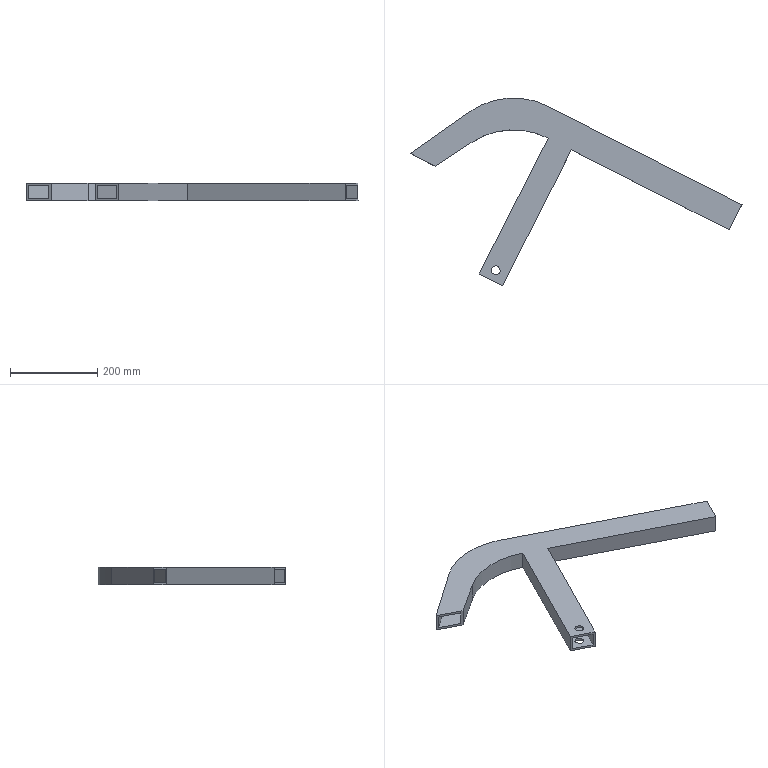Component | SolidWorks | FrameAssemblyDrawing11111-1_PartFrameCorner-1 | 1 solid | 30 faces | box 762.68 x 431.5 x 40 mm | volume 1076455 mm3 | plane 22 | cylinder 8 | commonest cylinder face diameters 20 x4 350 x2 360 x1 340 x1
STEP:
#1=COLOUR_RGB('',0.7922,0.8196,0.9333);
#2=FILL_AREA_STYLE_COLOUR('',#1);
#3=FILL_AREA_STYLE('',(#2));
#4=SURFACE_STYLE_FILL_AREA(#3);
#5=SURFACE_SIDE_STYLE('',(#4));
#6=SURFACE_STYLE_USAGE(.BOTH.,#5);
#7=PRESENTATION_STYLE_ASSIGNMENT((#6));
#8=CARTESIAN_POINT('',(-46.867,-24.103,40.983));
#9=VERTEX_POINT('',#8);
#10=CARTESIAN_POINT('',(-46.165,-24.459,40.983));
#11=VERTEX_POINT('',#10);
#12=CARTESIAN_POINT('',(-46.516,-24.281,40.983));
#13=DIRECTION('',(-0.,-0.,1.));
#14=DIRECTION('',(0.892,-0.4521,-0.));
#15=AXIS2_PLACEMENT_3D('',#12,#13,#14);
#16=CIRCLE('',#15,0.3937);
#17=EDGE_CURVE('',#9,#11,#16,.T.);
#18=ORIENTED_EDGE('',*,*,#17,.F.);
#19=CARTESIAN_POINT('',(-46.867,-24.103,41.18));
#20=VERTEX_POINT('',#19);
#21=CARTESIAN_POINT('',(-46.867,-24.103,40.983));
#22=DIRECTION('',(-0.,-0.,1.));
#23=VECTOR('',#22,39.37);
#24=LINE('',#21,#23);
#25=EDGE_CURVE('',#9,#20,#24,.T.);
#26=ORIENTED_EDGE('',*,*,#25,.T.);
#27=CARTESIAN_POINT('',(-46.165,-24.459,41.18));
#28=VERTEX_POINT('',#27);
#29=CARTESIAN_POINT('',(-46.516,-24.281,41.18));
#30=DIRECTION('',(-0.,-0.,1.));
#31=DIRECTION('',(0.892,-0.4521,-0.));
#32=AXIS2_PLACEMENT_3D('',#29,#30,#31);
#33=CIRCLE('',#32,0.3937);
#34=EDGE_CURVE('',#20,#28,#33,.T.);
#35=ORIENTED_EDGE('',*,*,#34,.T.);
#36=CARTESIAN_POINT('',(-46.165,-24.459,40.983));
#37=DIRECTION('',(-0.,-0.,1.));
#38=VECTOR('',#37,39.37);
#39=LINE('',#36,#38);
#40=EDGE_CURVE('',#11,#28,#39,.T.);
#41=ORIENTED_EDGE('',*,*,#40,.F.);
#42=EDGE_LOOP('',(#18,#26,#35,#41));
#43=FACE_OUTER_BOUND('',#42,.T.);
#44=CARTESIAN_POINT('',(-46.516,-24.281,40.983));
#45=DIRECTION('',(-0.,-0.,1.));
#46=DIRECTION('',(0.892,-0.4521,-0.));
#47=AXIS2_PLACEMENT_3D('',#44,#45,#46);
#48=CYLINDRICAL_SURFACE('',#47,0.3937);
#49=ADVANCED_FACE('',(#43),#48,.F.);
#50=CARTESIAN_POINT('',(-46.165,-24.459,42.361));
#51=VERTEX_POINT('',#50);
#52=CARTESIAN_POINT('',(-46.867,-24.103,42.361));
#53=VERTEX_POINT('',#52);
#54=CARTESIAN_POINT('',(-46.516,-24.281,42.361));
#55=DIRECTION('',(0.,0.,-1.));
#56=DIRECTION('',(-0.892,0.4521,0.));
#57=AXIS2_PLACEMENT_3D('',#54,#55,#56);
#58=CIRCLE('',#57,0.3937);
#59=EDGE_CURVE('',#51,#53,#58,.T.);
#60=ORIENTED_EDGE('',*,*,#59,.T.);
#61=CARTESIAN_POINT('',(-46.867,-24.103,42.558));
#62=VERTEX_POINT('',#61);
#63=CARTESIAN_POINT('',(-46.867,-24.103,40.983));
#64=DIRECTION('',(-0.,-0.,1.));
#65=VECTOR('',#64,39.37);
#66=LINE('',#63,#65);
#67=EDGE_CURVE('',#53,#62,#66,.T.);
#68=ORIENTED_EDGE('',*,*,#67,.T.);
#69=CARTESIAN_POINT('',(-46.165,-24.459,42.558));
#70=VERTEX_POINT('',#69);
#71=CARTESIAN_POINT('',(-46.516,-24.281,42.558));
#72=DIRECTION('',(-0.,-0.,1.));
#73=DIRECTION('',(0.892,-0.4521,-0.));
#74=AXIS2_PLACEMENT_3D('',#71,#72,#73);
#75=CIRCLE('',#74,0.3937);
#76=EDGE_CURVE('',#62,#70,#75,.T.);
#77=ORIENTED_EDGE('',*,*,#76,.T.);
#78=CARTESIAN_POINT('',(-46.165,-24.459,40.983));
#79=DIRECTION('',(-0.,-0.,1.));
#80=VECTOR('',#79,39.37);
#81=LINE('',#78,#80);
#82=EDGE_CURVE('',#51,#70,#81,.T.);
#83=ORIENTED_EDGE('',*,*,#82,.F.);
#84=EDGE_LOOP('',(#60,#68,#77,#83));
#85=FACE_OUTER_BOUND('',#84,.T.);
#86=CARTESIAN_POINT('',(-46.516,-24.281,40.983));
#87=DIRECTION('',(-0.,-0.,1.));
#88=DIRECTION('',(0.892,-0.4521,-0.));
#89=AXIS2_PLACEMENT_3D('',#86,#87,#88);
#90=CYLINDRICAL_SURFACE('',#89,0.3937);
#91=ADVANCED_FACE('',(#85),#90,.F.);
#92=CARTESIAN_POINT('',(-39.678,-13.402,40.983));
#93=VERTEX_POINT('',#92);
#94=CARTESIAN_POINT('',(-39.678,-13.402,42.558));
#95=VERTEX_POINT('',#94);
#96=CARTESIAN_POINT('',(-39.678,-13.402,40.983));
#97=DIRECTION('',(-0.,-0.,1.));
#98=VECTOR('',#97,39.37);
#99=LINE('',#96,#98);
#100=EDGE_CURVE('',#93,#95,#99,.T.);
#101=ORIENTED_EDGE('',*,*,#100,.F.);
#102=CARTESIAN_POINT('',(-25.406,-20.636,40.983));
#103=VERTEX_POINT('',#102);
#104=CARTESIAN_POINT('',(-41.785,-12.334,40.983));
#105=DIRECTION('',(0.892,-0.4521,-0.));
#106=VECTOR('',#105,39.37);
#107=LINE('',#104,#106);
#108=EDGE_CURVE('',#93,#103,#107,.T.);
#109=ORIENTED_EDGE('',*,*,#108,.T.);
#110=CARTESIAN_POINT('',(-25.406,-20.636,42.558));
#111=VERTEX_POINT('',#110);
#112=CARTESIAN_POINT('',(-25.406,-20.636,42.558));
#113=DIRECTION('',(0.,0.,-1.));
#114=VECTOR('',#113,39.37);
#115=LINE('',#112,#114);
#116=EDGE_CURVE('',#111,#103,#115,.T.);
#117=ORIENTED_EDGE('',*,*,#116,.F.);
#118=CARTESIAN_POINT('',(-41.785,-12.334,42.558));
#119=DIRECTION('',(0.892,-0.4521,-0.));
#120=VECTOR('',#119,39.37);
#121=LINE('',#118,#120);
#122=EDGE_CURVE('',#95,#111,#121,.T.);
#123=ORIENTED_EDGE('',*,*,#122,.F.);
#124=EDGE_LOOP('',(#101,#109,#117,#123));
#125=FACE_OUTER_BOUND('',#124,.T.);
#126=CARTESIAN_POINT('',(-41.785,-12.334,42.558));
#127=DIRECTION('',(0.4521,0.892,0.));
#128=DIRECTION('',(-0.892,0.4521,0.));
#129=AXIS2_PLACEMENT_3D('',#126,#127,#128);
#130=PLANE('',#129);
#131=ADVANCED_FACE('',(#125),#130,.F.);
#132=CARTESIAN_POINT('',(-54.273,-13.723,40.983));
#133=VERTEX_POINT('',#132);
#134=CARTESIAN_POINT('',(-51.991,-14.88,40.983));
#135=VERTEX_POINT('',#134);
#136=CARTESIAN_POINT('',(-54.273,-13.723,40.983));
#137=DIRECTION('',(0.892,-0.4521,-0.));
#138=VECTOR('',#137,39.37);
#139=LINE('',#136,#138);
#140=EDGE_CURVE('',#133,#135,#139,.T.);
#141=ORIENTED_EDGE('',*,*,#140,.T.);
#142=CARTESIAN_POINT('',(-51.991,-14.88,42.558));
#143=VERTEX_POINT('',#142);
#144=CARTESIAN_POINT('',(-51.991,-14.88,42.558));
#145=DIRECTION('',(0.,0.,-1.));
#146=VECTOR('',#145,39.37);
#147=LINE('',#144,#146);
#148=EDGE_CURVE('',#143,#135,#147,.T.);
#149=ORIENTED_EDGE('',*,*,#148,.F.);
#150=CARTESIAN_POINT('',(-54.273,-13.723,42.558));
#151=VERTEX_POINT('',#150);
#152=CARTESIAN_POINT('',(-54.273,-13.723,42.558));
#153=DIRECTION('',(0.892,-0.4521,-0.));
#154=VECTOR('',#153,39.37);
#155=LINE('',#152,#154);
#156=EDGE_CURVE('',#151,#143,#155,.T.);
#157=ORIENTED_EDGE('',*,*,#156,.F.);
#158=CARTESIAN_POINT('',(-54.273,-13.723,42.558));
#159=DIRECTION('',(0.,0.,-1.));
#160=VECTOR('',#159,39.37);
#161=LINE('',#158,#160);
#162=EDGE_CURVE('',#151,#133,#161,.T.);
#163=ORIENTED_EDGE('',*,*,#162,.T.);
#164=EDGE_LOOP('',(#141,#149,#157,#163));
#165=FACE_OUTER_BOUND('',#164,.T.);
#166=CARTESIAN_POINT('',(-54.074,-13.824,41.18));
#167=VERTEX_POINT('',#166);
#168=CARTESIAN_POINT('',(-52.194,-14.777,41.18));
#169=VERTEX_POINT('',#168);
#170=CARTESIAN_POINT('',(-46.077,-17.877,41.18));
#171=DIRECTION('',(0.892,-0.4521,-0.));
#172=VECTOR('',#171,39.37);
#173=LINE('',#170,#172);
#174=EDGE_CURVE('',#167,#169,#173,.T.);
#175=ORIENTED_EDGE('',*,*,#174,.F.);
#176=CARTESIAN_POINT('',(-54.074,-13.824,42.361));
#177=VERTEX_POINT('',#176);
#178=CARTESIAN_POINT('',(-54.074,-13.824,42.558));
#179=DIRECTION('',(0.,0.,-1.));
#180=VECTOR('',#179,39.37);
#181=LINE('',#178,#180);
#182=EDGE_CURVE('',#177,#167,#181,.T.);
#183=ORIENTED_EDGE('',*,*,#182,.F.);
#184=CARTESIAN_POINT('',(-52.194,-14.777,42.361));
#185=VERTEX_POINT('',#184);
#186=CARTESIAN_POINT('',(-46.077,-17.877,42.361));
#187=DIRECTION('',(0.892,-0.4521,-0.));
#188=VECTOR('',#187,39.37);
#189=LINE('',#186,#188);
#190=EDGE_CURVE('',#177,#185,#189,.T.);
#191=ORIENTED_EDGE('',*,*,#190,.T.);
#192=CARTESIAN_POINT('',(-52.194,-14.777,42.558));
#193=DIRECTION('',(0.,0.,-1.));
#194=VECTOR('',#193,39.37);
#195=LINE('',#192,#194);
#196=EDGE_CURVE('',#185,#169,#195,.T.);
#197=ORIENTED_EDGE('',*,*,#196,.T.);
#198=EDGE_LOOP('',(#175,#183,#191,#197));
#199=FACE_BOUND('',#198,.T.);
#200=CARTESIAN_POINT('',(-54.273,-13.723,42.558));
#201=DIRECTION('',(0.4521,0.892,0.));
#202=DIRECTION('',(-0.,-0.,1.));
#203=AXIS2_PLACEMENT_3D('',#200,#201,#202);
#204=PLANE('',#203);
#205=ADVANCED_FACE('',(#165,#199),#204,.F.);
#206=CARTESIAN_POINT('',(-24.247,-18.349,40.983));
#207=VERTEX_POINT('',#206);
#208=CARTESIAN_POINT('',(-24.247,-18.349,40.983));
#209=DIRECTION('',(0.4521,0.892,0.));
#210=VECTOR('',#209,39.37);
#211=LINE('',#208,#210);
#212=EDGE_CURVE('',#103,#207,#211,.T.);
#213=ORIENTED_EDGE('',*,*,#212,.T.);
#214=CARTESIAN_POINT('',(-24.247,-18.349,42.558));
#215=VERTEX_POINT('',#214);
#216=CARTESIAN_POINT('',(-24.247,-18.349,42.558));
#217=DIRECTION('',(0.,0.,-1.));
#218=VECTOR('',#217,39.37);
#219=LINE('',#216,#218);
#220=EDGE_CURVE('',#215,#207,#219,.T.);
#221=ORIENTED_EDGE('',*,*,#220,.F.);
#222=CARTESIAN_POINT('',(-24.247,-18.349,42.558));
#223=DIRECTION('',(0.4521,0.892,0.));
#224=VECTOR('',#223,39.37);
#225=LINE('',#222,#224);
#226=EDGE_CURVE('',#111,#215,#225,.T.);
#227=ORIENTED_EDGE('',*,*,#226,.F.);
#228=ORIENTED_EDGE('',*,*,#116,.T.);
#229=EDGE_LOOP('',(#213,#221,#227,#228));
#230=FACE_OUTER_BOUND('',#229,.T.);
#231=CARTESIAN_POINT('',(-25.317,-20.461,41.18));
#232=VERTEX_POINT('',#231);
#233=CARTESIAN_POINT('',(-24.336,-18.524,41.18));
#234=VERTEX_POINT('',#233);
#235=CARTESIAN_POINT('',(-27.361,-24.494,41.18));
#236=DIRECTION('',(0.4521,0.892,0.));
#237=VECTOR('',#236,39.37);
#238=LINE('',#235,#237);
#239=EDGE_CURVE('',#232,#234,#238,.T.);
#240=ORIENTED_EDGE('',*,*,#239,.F.);
#241=CARTESIAN_POINT('',(-25.317,-20.461,42.361));
#242=VERTEX_POINT('',#241);
#243=CARTESIAN_POINT('',(-25.317,-20.461,42.558));
#244=DIRECTION('',(0.,0.,-1.));
#245=VECTOR('',#244,39.37);
#246=LINE('',#243,#245);
#247=EDGE_CURVE('',#242,#232,#246,.T.);
#248=ORIENTED_EDGE('',*,*,#247,.F.);
#249=CARTESIAN_POINT('',(-24.336,-18.524,42.361));
#250=VERTEX_POINT('',#249);
#251=CARTESIAN_POINT('',(-27.361,-24.494,42.361));
#252=DIRECTION('',(0.4521,0.892,0.));
#253=VECTOR('',#252,39.37);
#254=LINE('',#251,#253);
#255=EDGE_CURVE('',#242,#250,#254,.T.);
#256=ORIENTED_EDGE('',*,*,#255,.T.);
#257=CARTESIAN_POINT('',(-24.336,-18.524,42.558));
#258=DIRECTION('',(0.,0.,-1.));
#259=VECTOR('',#258,39.37);
#260=LINE('',#257,#259);
#261=EDGE_CURVE('',#250,#234,#260,.T.);
#262=ORIENTED_EDGE('',*,*,#261,.T.);
#263=EDGE_LOOP('',(#240,#248,#256,#262));
#264=FACE_BOUND('',#263,.T.);
#265=CARTESIAN_POINT('',(-24.247,-18.349,42.558));
#266=DIRECTION('',(-0.892,0.4521,0.));
#267=DIRECTION('',(-0.,-0.,1.));
#268=AXIS2_PLACEMENT_3D('',#265,#266,#267);
#269=PLANE('',#268);
#270=ADVANCED_FACE('',(#230,#264),#269,.F.);
#271=CARTESIAN_POINT('',(-48.864,-9.946,40.983));
#272=VERTEX_POINT('',#271);
#273=CARTESIAN_POINT('',(-54.273,-13.723,40.983));
#274=DIRECTION('',(-0.8199,-0.5725,-0.));
#275=VECTOR('',#274,39.37);
#276=LINE('',#273,#275);
#277=EDGE_CURVE('',#272,#133,#276,.T.);
#278=ORIENTED_EDGE('',*,*,#277,.T.);
#279=ORIENTED_EDGE('',*,*,#162,.F.);
#280=CARTESIAN_POINT('',(-48.864,-9.946,42.558));
#281=VERTEX_POINT('',#280);
#282=CARTESIAN_POINT('',(-54.273,-13.723,42.558));
#283=DIRECTION('',(-0.8199,-0.5725,-0.));
#284=VECTOR('',#283,39.37);
#285=LINE('',#282,#284);
#286=EDGE_CURVE('',#281,#151,#285,.T.);
#287=ORIENTED_EDGE('',*,*,#286,.F.);
#288=CARTESIAN_POINT('',(-48.864,-9.946,42.558));
#289=DIRECTION('',(0.,0.,-1.));
#290=VECTOR('',#289,39.37);
#291=LINE('',#288,#290);
#292=EDGE_CURVE('',#281,#272,#291,.T.);
#293=ORIENTED_EDGE('',*,*,#292,.T.);
#294=EDGE_LOOP('',(#278,#279,#287,#293));
#295=FACE_OUTER_BOUND('',#294,.T.);
#296=CARTESIAN_POINT('',(-54.273,-13.723,42.558));
#297=DIRECTION('',(0.5725,-0.8199,-0.));
#298=DIRECTION('',(0.8199,0.5725,0.));
#299=AXIS2_PLACEMENT_3D('',#296,#297,#298);
#300=PLANE('',#299);
#301=ADVANCED_FACE('',(#295),#300,.F.);
#302=CARTESIAN_POINT('',(-48.664,-12.71,40.983));
#303=VERTEX_POINT('',#302);
#304=CARTESIAN_POINT('',(-51.991,-14.88,40.983));
#305=DIRECTION('',(0.8375,0.5464,0.));
#306=VECTOR('',#305,39.37);
#307=LINE('',#304,#306);
#308=EDGE_CURVE('',#135,#303,#307,.T.);
#309=ORIENTED_EDGE('',*,*,#308,.T.);
#310=CARTESIAN_POINT('',(-48.664,-12.71,42.558));
#311=VERTEX_POINT('',#310);
#312=CARTESIAN_POINT('',(-48.664,-12.71,42.558));
#313=DIRECTION('',(0.,0.,-1.));
#314=VECTOR('',#313,39.37);
#315=LINE('',#312,#314);
#316=EDGE_CURVE('',#311,#303,#315,.T.);
#317=ORIENTED_EDGE('',*,*,#316,.F.);
#318=CARTESIAN_POINT('',(-51.991,-14.88,42.558));
#319=DIRECTION('',(0.8375,0.5464,0.));
#320=VECTOR('',#319,39.37);
#321=LINE('',#318,#320);
#322=EDGE_CURVE('',#143,#311,#321,.T.);
#323=ORIENTED_EDGE('',*,*,#322,.F.);
#324=ORIENTED_EDGE('',*,*,#148,.T.);
#325=EDGE_LOOP('',(#309,#317,#323,#324));
#326=FACE_OUTER_BOUND('',#325,.T.);
#327=CARTESIAN_POINT('',(-51.991,-14.88,42.558));
#328=DIRECTION('',(-0.5464,0.8375,0.));
#329=DIRECTION('',(-0.8375,-0.5464,-0.));
#330=AXIS2_PLACEMENT_3D('',#327,#328,#329);
#331=PLANE('',#330);
#332=ADVANCED_FACE('',(#326),#331,.F.);
#333=CARTESIAN_POINT('',(-41.785,-12.334,40.983));
#334=VERTEX_POINT('',#333);
#335=CARTESIAN_POINT('',(-44.9,-18.48,40.983));
#336=DIRECTION('',(0.,0.,-1.));
#337=DIRECTION('',(-0.892,0.4521,0.));
#338=AXIS2_PLACEMENT_3D('',#335,#336,#337);
#339=CIRCLE('',#338,6.89);
#340=EDGE_CURVE('',#303,#334,#339,.T.);
#341=ORIENTED_EDGE('',*,*,#340,.T.);
#342=CARTESIAN_POINT('',(-41.785,-12.334,42.558));
#343=VERTEX_POINT('',#342);
#344=CARTESIAN_POINT('',(-41.785,-12.334,42.558));
#345=DIRECTION('',(0.,0.,-1.));
#346=VECTOR('',#345,39.37);
#347=LINE('',#344,#346);
#348=EDGE_CURVE('',#343,#334,#347,.T.);
#349=ORIENTED_EDGE('',*,*,#348,.F.);
#350=CARTESIAN_POINT('',(-44.9,-18.48,42.558));
#351=DIRECTION('',(0.,0.,-1.));
#352=DIRECTION('',(-0.892,0.4521,0.));
#353=AXIS2_PLACEMENT_3D('',#350,#351,#352);
#354=CIRCLE('',#353,6.89);
#355=EDGE_CURVE('',#311,#343,#354,.T.);
#356=ORIENTED_EDGE('',*,*,#355,.F.);
#357=ORIENTED_EDGE('',*,*,#316,.T.);
#358=EDGE_LOOP('',(#341,#349,#356,#357));
#359=FACE_OUTER_BOUND('',#358,.T.);
#360=CARTESIAN_POINT('',(-44.9,-18.48,42.558));
#361=DIRECTION('',(0.,0.,-1.));
#362=DIRECTION('',(-0.892,0.4521,0.));
#363=AXIS2_PLACEMENT_3D('',#360,#361,#362);
#364=CYLINDRICAL_SURFACE('',#363,6.89);
#365=ADVANCED_FACE('',(#359),#364,.F.);
#366=CARTESIAN_POINT('',(-41.805,-9.449,40.983));
#367=VERTEX_POINT('',#366);
#368=CARTESIAN_POINT('',(-41.805,-9.449,40.983));
#369=DIRECTION('',(-0.892,0.4521,0.));
#370=VECTOR('',#369,39.37);
#371=LINE('',#368,#370);
#372=EDGE_CURVE('',#207,#367,#371,.T.);
#373=ORIENTED_EDGE('',*,*,#372,.T.);
#374=CARTESIAN_POINT('',(-41.805,-9.449,42.558));
#375=VERTEX_POINT('',#374);
#376=CARTESIAN_POINT('',(-41.805,-9.449,42.558));
#377=DIRECTION('',(0.,0.,-1.));
#378=VECTOR('',#377,39.37);
#379=LINE('',#376,#378);
#380=EDGE_CURVE('',#375,#367,#379,.T.);
#381=ORIENTED_EDGE('',*,*,#380,.F.);
#382=CARTESIAN_POINT('',(-41.805,-9.449,42.558));
#383=DIRECTION('',(-0.892,0.4521,0.));
#384=VECTOR('',#383,39.37);
#385=LINE('',#382,#384);
#386=EDGE_CURVE('',#215,#375,#385,.T.);
#387=ORIENTED_EDGE('',*,*,#386,.F.);
#388=ORIENTED_EDGE('',*,*,#220,.T.);
#389=EDGE_LOOP('',(#373,#381,#387,#388));
#390=FACE_OUTER_BOUND('',#389,.T.);
#391=CARTESIAN_POINT('',(-41.805,-9.449,42.558));
#392=DIRECTION('',(-0.4521,-0.892,-0.));
#393=DIRECTION('',(0.,0.,-1.));
#394=AXIS2_PLACEMENT_3D('',#391,#392,#393);
#395=PLANE('',#394);
#396=ADVANCED_FACE('',(#390),#395,.F.);
#397=CARTESIAN_POINT('',(-44.92,-15.595,40.983));
#398=DIRECTION('',(-0.,-0.,1.));
#399=DIRECTION('',(-0.892,0.4521,0.));
#400=AXIS2_PLACEMENT_3D('',#397,#398,#399);
#401=CIRCLE('',#400,6.89);
#402=EDGE_CURVE('',#367,#272,#401,.T.);
#403=ORIENTED_EDGE('',*,*,#402,.T.);
#404=ORIENTED_EDGE('',*,*,#292,.F.);
#405=CARTESIAN_POINT('',(-44.92,-15.595,42.558));
#406=DIRECTION('',(-0.,-0.,1.));
#407=DIRECTION('',(-0.892,0.4521,0.));
#408=AXIS2_PLACEMENT_3D('',#405,#406,#407);
#409=CIRCLE('',#408,6.89);
#410=EDGE_CURVE('',#375,#281,#409,.T.);
#411=ORIENTED_EDGE('',*,*,#410,.F.);
#412=ORIENTED_EDGE('',*,*,#380,.T.);
#413=EDGE_LOOP('',(#403,#404,#411,#412));
#414=FACE_OUTER_BOUND('',#413,.T.);
#415=CARTESIAN_POINT('',(-44.92,-15.595,42.558));
#416=DIRECTION('',(0.,0.,-1.));
#417=DIRECTION('',(-0.892,0.4521,0.));
#418=AXIS2_PLACEMENT_3D('',#415,#416,#417);
#419=CYLINDRICAL_SURFACE('',#418,6.89);
#420=ADVANCED_FACE('',(#414),#419,.T.);
#421=CARTESIAN_POINT('',(-46.516,-24.281,42.558));
#422=DIRECTION('',(-0.,-0.,1.));
#423=DIRECTION('',(0.892,-0.4521,-0.));
#424=AXIS2_PLACEMENT_3D('',#421,#422,#423);
#425=CIRCLE('',#424,0.3937);
#426=EDGE_CURVE('',#70,#62,#425,.T.);
#427=ORIENTED_EDGE('',*,*,#426,.F.);
#428=ORIENTED_EDGE('',*,*,#76,.F.);
#429=EDGE_LOOP('',(#427,#428));
#430=FACE_BOUND('',#429,.T.);
#431=ORIENTED_EDGE('',*,*,#286,.T.);
#432=ORIENTED_EDGE('',*,*,#156,.T.);
#433=ORIENTED_EDGE('',*,*,#322,.T.);
#434=ORIENTED_EDGE('',*,*,#355,.T.);
#435=CARTESIAN_POINT('',(-48.015,-24.625,42.558));
#436=VERTEX_POINT('',#435);
#437=CARTESIAN_POINT('',(-48.015,-24.625,42.558));
#438=DIRECTION('',(0.4521,0.892,0.));
#439=VECTOR('',#438,39.37);
#440=LINE('',#437,#439);
#441=EDGE_CURVE('',#436,#343,#440,.T.);
#442=ORIENTED_EDGE('',*,*,#441,.F.);
#443=CARTESIAN_POINT('',(-45.908,-25.693,42.558));
#444=VERTEX_POINT('',#443);
#445=CARTESIAN_POINT('',(-48.015,-24.625,42.558));
#446=DIRECTION('',(-0.892,0.4521,0.));
#447=VECTOR('',#446,39.37);
#448=LINE('',#445,#447);
#449=EDGE_CURVE('',#444,#436,#448,.T.);
#450=ORIENTED_EDGE('',*,*,#449,.F.);
#451=CARTESIAN_POINT('',(-45.908,-25.693,42.558));
#452=DIRECTION('',(0.4521,0.892,0.));
#453=VECTOR('',#452,39.37);
#454=LINE('',#451,#453);
#455=EDGE_CURVE('',#444,#95,#454,.T.);
#456=ORIENTED_EDGE('',*,*,#455,.T.);
#457=ORIENTED_EDGE('',*,*,#122,.T.);
#458=ORIENTED_EDGE('',*,*,#226,.T.);
#459=ORIENTED_EDGE('',*,*,#386,.T.);
#460=ORIENTED_EDGE('',*,*,#410,.T.);
#461=EDGE_LOOP('',(#431,#432,#433,#434,#442,#450,#456,#457,#458,#459,#460));
#462=FACE_OUTER_BOUND('',#461,.T.);
#463=CARTESIAN_POINT('',(-44.92,-15.595,42.558));
#464=DIRECTION('',(0.,0.,-1.));
#465=DIRECTION('',(-0.892,0.4521,0.));
#466=AXIS2_PLACEMENT_3D('',#463,#464,#465);
#467=PLANE('',#466);
#468=ADVANCED_FACE('',(#430,#462),#467,.F.);
#469=CARTESIAN_POINT('',(-46.516,-24.281,40.983));
#470=DIRECTION('',(-0.,-0.,1.));
#471=DIRECTION('',(0.892,-0.4521,-0.));
#472=AXIS2_PLACEMENT_3D('',#469,#470,#471);
#473=CIRCLE('',#472,0.3937);
#474=EDGE_CURVE('',#11,#9,#473,.T.);
#475=ORIENTED_EDGE('',*,*,#474,.T.);
#476=ORIENTED_EDGE('',*,*,#17,.T.);
#477=EDGE_LOOP('',(#475,#476));
#478=FACE_BOUND('',#477,.T.);
#479=ORIENTED_EDGE('',*,*,#277,.F.);
#480=ORIENTED_EDGE('',*,*,#402,.F.);
#481=ORIENTED_EDGE('',*,*,#372,.F.);
#482=ORIENTED_EDGE('',*,*,#212,.F.);
#483=ORIENTED_EDGE('',*,*,#108,.F.);
#484=CARTESIAN_POINT('',(-45.908,-25.693,40.983));
#485=VERTEX_POINT('',#484);
#486=CARTESIAN_POINT('',(-45.908,-25.693,40.983));
#487=DIRECTION('',(0.4521,0.892,0.));
#488=VECTOR('',#487,39.37);
#489=LINE('',#486,#488);
#490=EDGE_CURVE('',#485,#93,#489,.T.);
#491=ORIENTED_EDGE('',*,*,#490,.F.);
#492=CARTESIAN_POINT('',(-48.015,-24.625,40.983));
#493=VERTEX_POINT('',#492);
#494=CARTESIAN_POINT('',(-48.015,-24.625,40.983));
#495=DIRECTION('',(0.892,-0.4521,-0.));
#496=VECTOR('',#495,39.37);
#497=LINE('',#494,#496);
#498=EDGE_CURVE('',#493,#485,#497,.T.);
#499=ORIENTED_EDGE('',*,*,#498,.F.);
#500=CARTESIAN_POINT('',(-48.015,-24.625,40.983));
#501=DIRECTION('',(0.4521,0.892,0.));
#502=VECTOR('',#501,39.37);
#503=LINE('',#500,#502);
#504=EDGE_CURVE('',#493,#334,#503,.T.);
#505=ORIENTED_EDGE('',*,*,#504,.T.);
#506=ORIENTED_EDGE('',*,*,#340,.F.);
#507=ORIENTED_EDGE('',*,*,#308,.F.);
#508=ORIENTED_EDGE('',*,*,#140,.F.);
#509=EDGE_LOOP('',(#479,#480,#481,#482,#483,#491,#499,#505,#506,#507,#508));
#510=FACE_OUTER_BOUND('',#509,.T.);
#511=CARTESIAN_POINT('',(-44.92,-15.595,40.983));
#512=DIRECTION('',(0.,0.,-1.));
#513=DIRECTION('',(-0.892,0.4521,0.));
#514=AXIS2_PLACEMENT_3D('',#511,#512,#513);
#515=PLANE('',#514);
#516=ADVANCED_FACE('',(#478,#510),#515,.T.);
#517=CARTESIAN_POINT('',(-48.752,-10.107,41.18));
#518=VERTEX_POINT('',#517);
#519=CARTESIAN_POINT('',(-48.752,-10.107,41.18));
#520=DIRECTION('',(-0.8199,-0.5725,-0.));
#521=VECTOR('',#520,39.37);
#522=LINE('',#519,#521);
#523=EDGE_CURVE('',#518,#167,#522,.T.);
#524=ORIENTED_EDGE('',*,*,#523,.F.);
#525=CARTESIAN_POINT('',(-48.752,-10.107,42.361));
#526=VERTEX_POINT('',#525);
#527=CARTESIAN_POINT('',(-48.752,-10.107,42.558));
#528=DIRECTION('',(0.,0.,-1.));
#529=VECTOR('',#528,39.37);
#530=LINE('',#527,#529);
#531=EDGE_CURVE('',#526,#518,#530,.T.);
#532=ORIENTED_EDGE('',*,*,#531,.F.);
#533=CARTESIAN_POINT('',(-48.752,-10.107,42.361));
#534=DIRECTION('',(-0.8199,-0.5725,-0.));
#535=VECTOR('',#534,39.37);
#536=LINE('',#533,#535);
#537=EDGE_CURVE('',#526,#177,#536,.T.);
#538=ORIENTED_EDGE('',*,*,#537,.T.);
#539=ORIENTED_EDGE('',*,*,#182,.T.);
#540=EDGE_LOOP('',(#524,#532,#538,#539));
#541=FACE_OUTER_BOUND('',#540,.T.);
#542=CARTESIAN_POINT('',(-54.161,-13.884,42.558));
#543=DIRECTION('',(0.5725,-0.8199,-0.));
#544=DIRECTION('',(0.8199,0.5725,0.));
#545=AXIS2_PLACEMENT_3D('',#542,#543,#544);
#546=PLANE('',#545);
#547=ADVANCED_FACE('',(#541),#546,.T.);
#548=CARTESIAN_POINT('',(-48.772,-12.545,41.18));
#549=VERTEX_POINT('',#548);
#550=CARTESIAN_POINT('',(-47.466,-11.692,41.18));
#551=DIRECTION('',(0.8375,0.5464,0.));
#552=VECTOR('',#551,39.37);
#553=LINE('',#550,#552);
#554=EDGE_CURVE('',#169,#549,#553,.T.);
#555=ORIENTED_EDGE('',*,*,#554,.F.);
#556=ORIENTED_EDGE('',*,*,#196,.F.);
#557=CARTESIAN_POINT('',(-48.772,-12.545,42.361));
#558=VERTEX_POINT('',#557);
#559=CARTESIAN_POINT('',(-47.466,-11.692,42.361));
#560=DIRECTION('',(0.8375,0.5464,0.));
#561=VECTOR('',#560,39.37);
#562=LINE('',#559,#561);
#563=EDGE_CURVE('',#185,#558,#562,.T.);
#564=ORIENTED_EDGE('',*,*,#563,.T.);
#565=CARTESIAN_POINT('',(-48.772,-12.545,42.558));
#566=DIRECTION('',(0.,0.,-1.));
#567=VECTOR('',#566,39.37);
#568=LINE('',#565,#567);
#569=EDGE_CURVE('',#558,#549,#568,.T.);
#570=ORIENTED_EDGE('',*,*,#569,.T.);
#571=EDGE_LOOP('',(#555,#556,#564,#570));
#572=FACE_OUTER_BOUND('',#571,.T.);
#573=CARTESIAN_POINT('',(-52.098,-14.715,42.558));
#574=DIRECTION('',(-0.5464,0.8375,0.));
#575=DIRECTION('',(-0.8375,-0.5464,-0.));
#576=AXIS2_PLACEMENT_3D('',#573,#574,#575);
#577=PLANE('',#576);
#578=ADVANCED_FACE('',(#572),#577,.T.);
#579=CARTESIAN_POINT('',(-41.696,-12.159,41.18));
#580=VERTEX_POINT('',#579);
#581=CARTESIAN_POINT('',(-44.9,-18.48,41.18));
#582=DIRECTION('',(0.,0.,-1.));
#583=DIRECTION('',(-0.892,0.4521,0.));
#584=AXIS2_PLACEMENT_3D('',#581,#582,#583);
#585=CIRCLE('',#584,7.087);
#586=EDGE_CURVE('',#549,#580,#585,.T.);
#587=ORIENTED_EDGE('',*,*,#586,.F.);
#588=ORIENTED_EDGE('',*,*,#569,.F.);
#589=CARTESIAN_POINT('',(-41.696,-12.159,42.361));
#590=VERTEX_POINT('',#589);
#591=CARTESIAN_POINT('',(-44.9,-18.48,42.361));
#592=DIRECTION('',(0.,0.,-1.));
#593=DIRECTION('',(-0.892,0.4521,0.));
#594=AXIS2_PLACEMENT_3D('',#591,#592,#593);
#595=CIRCLE('',#594,7.087);
#596=EDGE_CURVE('',#558,#590,#595,.T.);
#597=ORIENTED_EDGE('',*,*,#596,.T.);
#598=CARTESIAN_POINT('',(-41.696,-12.159,42.558));
#599=DIRECTION('',(0.,0.,-1.));
#600=VECTOR('',#599,39.37);
#601=LINE('',#598,#600);
#602=EDGE_CURVE('',#590,#580,#601,.T.);
#603=ORIENTED_EDGE('',*,*,#602,.T.);
#604=EDGE_LOOP('',(#587,#588,#597,#603));
#605=FACE_OUTER_BOUND('',#604,.T.);
#606=CARTESIAN_POINT('',(-44.9,-18.48,42.558));
#607=DIRECTION('',(0.,0.,-1.));
#608=DIRECTION('',(-0.892,0.4521,0.));
#609=AXIS2_PLACEMENT_3D('',#606,#607,#608);
#610=CYLINDRICAL_SURFACE('',#609,7.087);
#611=ADVANCED_FACE('',(#605),#610,.T.);
#612=CARTESIAN_POINT('',(-42.875,-11.561,41.18));
#613=DIRECTION('',(0.892,-0.4521,-0.));
#614=VECTOR('',#613,39.37);
#615=LINE('',#612,#614);
#616=EDGE_CURVE('',#580,#232,#615,.T.);
#617=ORIENTED_EDGE('',*,*,#616,.F.);
#618=ORIENTED_EDGE('',*,*,#602,.F.);
#619=CARTESIAN_POINT('',(-42.875,-11.561,42.361));
#620=DIRECTION('',(0.892,-0.4521,-0.));
#621=VECTOR('',#620,39.37);
#622=LINE('',#619,#621);
#623=EDGE_CURVE('',#590,#242,#622,.T.);
#624=ORIENTED_EDGE('',*,*,#623,.T.);
#625=ORIENTED_EDGE('',*,*,#247,.T.);
#626=EDGE_LOOP('',(#617,#618,#624,#625));
#627=FACE_OUTER_BOUND('',#626,.T.);
#628=CARTESIAN_POINT('',(-41.696,-12.159,42.558));
#629=DIRECTION('',(0.4521,0.892,0.));
#630=DIRECTION('',(-0.892,0.4521,0.));
#631=AXIS2_PLACEMENT_3D('',#628,#629,#630);
#632=PLANE('',#631);
#633=ADVANCED_FACE('',(#627),#632,.T.);
#634=CARTESIAN_POINT('',(-41.894,-9.625,41.18));
#635=VERTEX_POINT('',#634);
#636=CARTESIAN_POINT('',(-41.894,-9.625,41.18));
#637=DIRECTION('',(-0.892,0.4521,0.));
#638=VECTOR('',#637,39.37);
#639=LINE('',#636,#638);
#640=EDGE_CURVE('',#234,#635,#639,.T.);
#641=ORIENTED_EDGE('',*,*,#640,.F.);
#642=ORIENTED_EDGE('',*,*,#261,.F.);
#643=CARTESIAN_POINT('',(-41.894,-9.625,42.361));
#644=VERTEX_POINT('',#643);
#645=CARTESIAN_POINT('',(-41.894,-9.625,42.361));
#646=DIRECTION('',(-0.892,0.4521,0.));
#647=VECTOR('',#646,39.37);
#648=LINE('',#645,#647);
#649=EDGE_CURVE('',#250,#644,#648,.T.);
#650=ORIENTED_EDGE('',*,*,#649,.T.);
#651=CARTESIAN_POINT('',(-41.894,-9.625,42.558));
#652=DIRECTION('',(0.,0.,-1.));
#653=VECTOR('',#652,39.37);
#654=LINE('',#651,#653);
#655=EDGE_CURVE('',#644,#635,#654,.T.);
#656=ORIENTED_EDGE('',*,*,#655,.T.);
#657=EDGE_LOOP('',(#641,#642,#650,#656));
#658=FACE_OUTER_BOUND('',#657,.T.);
#659=CARTESIAN_POINT('',(-41.894,-9.625,42.558));
#660=DIRECTION('',(-0.4521,-0.892,-0.));
#661=DIRECTION('',(0.,0.,-1.));
#662=AXIS2_PLACEMENT_3D('',#659,#660,#661);
#663=PLANE('',#662);
#664=ADVANCED_FACE('',(#658),#663,.T.);
#665=CARTESIAN_POINT('',(-44.92,-15.595,41.18));
#666=DIRECTION('',(-0.,-0.,1.));
#667=DIRECTION('',(-0.892,0.4521,0.));
#668=AXIS2_PLACEMENT_3D('',#665,#666,#667);
#669=CIRCLE('',#668,6.693);
#670=EDGE_CURVE('',#635,#518,#669,.T.);
#671=ORIENTED_EDGE('',*,*,#670,.F.);
#672=ORIENTED_EDGE('',*,*,#655,.F.);
#673=CARTESIAN_POINT('',(-44.92,-15.595,42.361));
#674=DIRECTION('',(-0.,-0.,1.));
#675=DIRECTION('',(-0.892,0.4521,0.));
#676=AXIS2_PLACEMENT_3D('',#673,#674,#675);
#677=CIRCLE('',#676,6.693);
#678=EDGE_CURVE('',#644,#526,#677,.T.);
#679=ORIENTED_EDGE('',*,*,#678,.T.);
#680=ORIENTED_EDGE('',*,*,#531,.T.);
#681=EDGE_LOOP('',(#671,#672,#679,#680));
#682=FACE_OUTER_BOUND('',#681,.T.);
#683=CARTESIAN_POINT('',(-44.92,-15.595,42.558));
#684=DIRECTION('',(0.,0.,-1.));
#685=DIRECTION('',(-0.892,0.4521,0.));
#686=AXIS2_PLACEMENT_3D('',#683,#684,#685);
#687=CYLINDRICAL_SURFACE('',#686,6.693);
#688=ADVANCED_FACE('',(#682),#687,.F.);
#689=ORIENTED_EDGE('',*,*,#537,.F.);
#690=ORIENTED_EDGE('',*,*,#678,.F.);
#691=ORIENTED_EDGE('',*,*,#649,.F.);
#692=ORIENTED_EDGE('',*,*,#255,.F.);
#693=ORIENTED_EDGE('',*,*,#623,.F.);
#694=ORIENTED_EDGE('',*,*,#596,.F.);
#695=ORIENTED_EDGE('',*,*,#563,.F.);
#696=ORIENTED_EDGE('',*,*,#190,.F.);
#697=EDGE_LOOP('',(#689,#690,#691,#692,#693,#694,#695,#696));
#698=FACE_OUTER_BOUND('',#697,.T.);
#699=CARTESIAN_POINT('',(-44.92,-15.595,42.361));
#700=DIRECTION('',(0.,0.,-1.));
#701=DIRECTION('',(-0.892,0.4521,0.));
#702=AXIS2_PLACEMENT_3D('',#699,#700,#701);
#703=PLANE('',#702);
#704=ADVANCED_FACE('',(#698),#703,.T.);
#705=ORIENTED_EDGE('',*,*,#523,.T.);
#706=ORIENTED_EDGE('',*,*,#174,.T.);
#707=ORIENTED_EDGE('',*,*,#554,.T.);
#708=ORIENTED_EDGE('',*,*,#586,.T.);
#709=ORIENTED_EDGE('',*,*,#616,.T.);
#710=ORIENTED_EDGE('',*,*,#239,.T.);
#711=ORIENTED_EDGE('',*,*,#640,.T.);
#712=ORIENTED_EDGE('',*,*,#670,.T.);
#713=EDGE_LOOP('',(#705,#706,#707,#708,#709,#710,#711,#712));
#714=FACE_OUTER_BOUND('',#713,.T.);
#715=CARTESIAN_POINT('',(-44.92,-15.595,41.18));
#716=DIRECTION('',(0.,0.,-1.));
#717=DIRECTION('',(-0.892,0.4521,0.));
#718=AXIS2_PLACEMENT_3D('',#715,#716,#717);
#719=PLANE('',#718);
#720=ADVANCED_FACE('',(#714),#719,.F.);
#721=CARTESIAN_POINT('',(-48.015,-24.625,40.983));
#722=DIRECTION('',(0.,0.,-1.));
#723=VECTOR('',#722,39.37);
#724=LINE('',#721,#723);
#725=EDGE_CURVE('',#436,#493,#724,.T.);
#726=ORIENTED_EDGE('',*,*,#725,.T.);
#727=ORIENTED_EDGE('',*,*,#498,.T.);
#728=CARTESIAN_POINT('',(-45.908,-25.693,40.983));
#729=DIRECTION('',(-0.,-0.,1.));
#730=VECTOR('',#729,39.37);
#731=LINE('',#728,#730);
#732=EDGE_CURVE('',#485,#444,#731,.T.);
#733=ORIENTED_EDGE('',*,*,#732,.T.);
#734=ORIENTED_EDGE('',*,*,#449,.T.);
#735=EDGE_LOOP('',(#726,#727,#733,#734));
#736=FACE_OUTER_BOUND('',#735,.T.);
#737=CARTESIAN_POINT('',(-47.839,-24.714,42.361));
#738=VERTEX_POINT('',#737);
#739=CARTESIAN_POINT('',(-47.839,-24.714,41.18));
#740=VERTEX_POINT('',#739);
#741=CARTESIAN_POINT('',(-47.839,-24.714,41.18));
#742=DIRECTION('',(0.,0.,-1.));
#743=VECTOR('',#742,39.37);
#744=LINE('',#741,#743);
#745=EDGE_CURVE('',#738,#740,#744,.T.);
#746=ORIENTED_EDGE('',*,*,#745,.F.);
#747=CARTESIAN_POINT('',(-46.083,-25.604,42.361));
#748=VERTEX_POINT('',#747);
#749=CARTESIAN_POINT('',(-47.839,-24.714,42.361));
#750=DIRECTION('',(-0.892,0.4521,0.));
#751=VECTOR('',#750,39.37);
#752=LINE('',#749,#751);
#753=EDGE_CURVE('',#748,#738,#752,.T.);
#754=ORIENTED_EDGE('',*,*,#753,.F.);
#755=CARTESIAN_POINT('',(-46.083,-25.604,41.18));
#756=VERTEX_POINT('',#755);
#757=CARTESIAN_POINT('',(-46.083,-25.604,41.18));
#758=DIRECTION('',(-0.,-0.,1.));
#759=VECTOR('',#758,39.37);
#760=LINE('',#757,#759);
#761=EDGE_CURVE('',#756,#748,#760,.T.);
#762=ORIENTED_EDGE('',*,*,#761,.F.);
#763=CARTESIAN_POINT('',(-47.839,-24.714,41.18));
#764=DIRECTION('',(0.892,-0.4521,-0.));
#765=VECTOR('',#764,39.37);
#766=LINE('',#763,#765);
#767=EDGE_CURVE('',#740,#756,#766,.T.);
#768=ORIENTED_EDGE('',*,*,#767,.F.);
#769=EDGE_LOOP('',(#746,#754,#762,#768));
#770=FACE_BOUND('',#769,.T.);
#771=CARTESIAN_POINT('',(-77.289,-9.787,40.983));
#772=DIRECTION('',(0.4521,0.892,0.));
#773=DIRECTION('',(-0.,-0.,1.));
#774=AXIS2_PLACEMENT_3D('',#771,#772,#773);
#775=PLANE('',#774);
#776=ADVANCED_FACE('',(#736,#770),#775,.F.);
#777=ORIENTED_EDGE('',*,*,#348,.T.);
#778=ORIENTED_EDGE('',*,*,#504,.F.);
#779=ORIENTED_EDGE('',*,*,#725,.F.);
#780=ORIENTED_EDGE('',*,*,#441,.T.);
#781=EDGE_LOOP('',(#777,#778,#779,#780));
#782=FACE_OUTER_BOUND('',#781,.T.);
#783=CARTESIAN_POINT('',(-48.015,-24.625,40.983));
#784=DIRECTION('',(0.892,-0.4521,-0.));
#785=DIRECTION('',(0.4521,0.892,0.));
#786=AXIS2_PLACEMENT_3D('',#783,#784,#785);
#787=PLANE('',#786);
#788=ADVANCED_FACE('',(#782),#787,.F.);
#789=ORIENTED_EDGE('',*,*,#100,.T.);
#790=ORIENTED_EDGE('',*,*,#455,.F.);
#791=ORIENTED_EDGE('',*,*,#732,.F.);
#792=ORIENTED_EDGE('',*,*,#490,.T.);
#793=EDGE_LOOP('',(#789,#790,#791,#792));
#794=FACE_OUTER_BOUND('',#793,.T.);
#795=CARTESIAN_POINT('',(-45.908,-25.693,40.983));
#796=DIRECTION('',(-0.892,0.4521,0.));
#797=DIRECTION('',(-0.4521,-0.892,-0.));
#798=AXIS2_PLACEMENT_3D('',#795,#796,#797);
#799=PLANE('',#798);
#800=ADVANCED_FACE('',(#794),#799,.F.);
#801=CARTESIAN_POINT('',(-41.609,-12.423,42.361));
#802=VERTEX_POINT('',#801);
#803=CARTESIAN_POINT('',(-41.609,-12.423,41.18));
#804=VERTEX_POINT('',#803);
#805=CARTESIAN_POINT('',(-41.609,-12.423,41.18));
#806=DIRECTION('',(0.,0.,-1.));
#807=VECTOR('',#806,39.37);
#808=LINE('',#805,#807);
#809=EDGE_CURVE('',#802,#804,#808,.T.);
#810=ORIENTED_EDGE('',*,*,#809,.F.);
#811=CARTESIAN_POINT('',(-47.839,-24.714,42.361));
#812=DIRECTION('',(0.4521,0.892,0.));
#813=VECTOR('',#812,39.37);
#814=LINE('',#811,#813);
#815=EDGE_CURVE('',#738,#802,#814,.T.);
#816=ORIENTED_EDGE('',*,*,#815,.F.);
#817=ORIENTED_EDGE('',*,*,#745,.T.);
#818=CARTESIAN_POINT('',(-47.839,-24.714,41.18));
#819=DIRECTION('',(0.4521,0.892,0.));
#820=VECTOR('',#819,39.37);
#821=LINE('',#818,#820);
#822=EDGE_CURVE('',#740,#804,#821,.T.);
#823=ORIENTED_EDGE('',*,*,#822,.T.);
#824=EDGE_LOOP('',(#810,#816,#817,#823));
#825=FACE_OUTER_BOUND('',#824,.T.);
#826=CARTESIAN_POINT('',(-47.839,-24.714,41.18));
#827=DIRECTION('',(0.892,-0.4521,-0.));
#828=DIRECTION('',(0.4521,0.892,0.));
#829=AXIS2_PLACEMENT_3D('',#826,#827,#828);
#830=PLANE('',#829);
#831=ADVANCED_FACE('',(#825),#830,.T.);
#832=CARTESIAN_POINT('',(-46.516,-24.281,41.18));
#833=DIRECTION('',(-0.,-0.,1.));
#834=DIRECTION('',(0.892,-0.4521,-0.));
#835=AXIS2_PLACEMENT_3D('',#832,#833,#834);
#836=CIRCLE('',#835,0.3937);
#837=EDGE_CURVE('',#28,#20,#836,.T.);
#838=ORIENTED_EDGE('',*,*,#837,.F.);
#839=ORIENTED_EDGE('',*,*,#34,.F.);
#840=EDGE_LOOP('',(#838,#839));
#841=FACE_BOUND('',#840,.T.);
#842=CARTESIAN_POINT('',(-39.853,-13.313,41.18));
#843=VERTEX_POINT('',#842);
#844=CARTESIAN_POINT('',(-41.609,-12.423,41.18));
#845=DIRECTION('',(0.892,-0.4521,-0.));
#846=VECTOR('',#845,39.37);
#847=LINE('',#844,#846);
#848=EDGE_CURVE('',#804,#843,#847,.T.);
#849=ORIENTED_EDGE('',*,*,#848,.F.);
#850=ORIENTED_EDGE('',*,*,#822,.F.);
#851=ORIENTED_EDGE('',*,*,#767,.T.);
#852=CARTESIAN_POINT('',(-46.083,-25.604,41.18));
#853=DIRECTION('',(0.4521,0.892,0.));
#854=VECTOR('',#853,39.37);
#855=LINE('',#852,#854);
#856=EDGE_CURVE('',#756,#843,#855,.T.);
#857=ORIENTED_EDGE('',*,*,#856,.T.);
#858=EDGE_LOOP('',(#849,#850,#851,#857));
#859=FACE_OUTER_BOUND('',#858,.T.);
#860=CARTESIAN_POINT('',(-47.839,-24.714,41.18));
#861=DIRECTION('',(-0.,-0.,1.));
#862=DIRECTION('',(0.892,-0.4521,-0.));
#863=AXIS2_PLACEMENT_3D('',#860,#861,#862);
#864=PLANE('',#863);
#865=ADVANCED_FACE('',(#841,#859),#864,.T.);
#866=CARTESIAN_POINT('',(-39.853,-13.313,42.361));
#867=VERTEX_POINT('',#866);
#868=CARTESIAN_POINT('',(-39.853,-13.313,41.18));
#869=DIRECTION('',(-0.,-0.,1.));
#870=VECTOR('',#869,39.37);
#871=LINE('',#868,#870);
#872=EDGE_CURVE('',#843,#867,#871,.T.);
#873=ORIENTED_EDGE('',*,*,#872,.F.);
#874=ORIENTED_EDGE('',*,*,#856,.F.);
#875=ORIENTED_EDGE('',*,*,#761,.T.);
#876=CARTESIAN_POINT('',(-46.083,-25.604,42.361));
#877=DIRECTION('',(0.4521,0.892,0.));
#878=VECTOR('',#877,39.37);
#879=LINE('',#876,#878);
#880=EDGE_CURVE('',#748,#867,#879,.T.);
#881=ORIENTED_EDGE('',*,*,#880,.T.);
#882=EDGE_LOOP('',(#873,#874,#875,#881));
#883=FACE_OUTER_BOUND('',#882,.T.);
#884=CARTESIAN_POINT('',(-46.083,-25.604,41.18));
#885=DIRECTION('',(-0.892,0.4521,0.));
#886=DIRECTION('',(-0.4521,-0.892,-0.));
#887=AXIS2_PLACEMENT_3D('',#884,#885,#886);
#888=PLANE('',#887);
#889=ADVANCED_FACE('',(#883),#888,.T.);
#890=ORIENTED_EDGE('',*,*,#59,.F.);
#891=CARTESIAN_POINT('',(-46.516,-24.281,42.361));
#892=DIRECTION('',(0.,0.,-1.));
#893=DIRECTION('',(-0.892,0.4521,0.));
#894=AXIS2_PLACEMENT_3D('',#891,#892,#893);
#895=CIRCLE('',#894,0.3937);
#896=EDGE_CURVE('',#53,#51,#895,.T.);
#897=ORIENTED_EDGE('',*,*,#896,.F.);
#898=EDGE_LOOP('',(#890,#897));
#899=FACE_BOUND('',#898,.T.);
#900=CARTESIAN_POINT('',(-41.609,-12.423,42.361));
#901=DIRECTION('',(-0.892,0.4521,0.));
#902=VECTOR('',#901,39.37);
#903=LINE('',#900,#902);
#904=EDGE_CURVE('',#867,#802,#903,.T.);
#905=ORIENTED_EDGE('',*,*,#904,.F.);
#906=ORIENTED_EDGE('',*,*,#880,.F.);
#907=ORIENTED_EDGE('',*,*,#753,.T.);
#908=ORIENTED_EDGE('',*,*,#815,.T.);
#909=EDGE_LOOP('',(#905,#906,#907,#908));
#910=FACE_OUTER_BOUND('',#909,.T.);
#911=CARTESIAN_POINT('',(-47.839,-24.714,42.361));
#912=DIRECTION('',(0.,0.,-1.));
#913=DIRECTION('',(-0.892,0.4521,0.));
#914=AXIS2_PLACEMENT_3D('',#911,#912,#913);
#915=PLANE('',#914);
#916=ADVANCED_FACE('',(#899,#910),#915,.T.);
#917=ORIENTED_EDGE('',*,*,#904,.T.);
#918=ORIENTED_EDGE('',*,*,#809,.T.);
#919=ORIENTED_EDGE('',*,*,#848,.T.);
#920=ORIENTED_EDGE('',*,*,#872,.T.);
#921=EDGE_LOOP('',(#917,#918,#919,#920));
#922=FACE_OUTER_BOUND('',#921,.T.);
#923=CARTESIAN_POINT('',(-41.785,-12.334,42.558));
#924=DIRECTION('',(0.4521,0.892,0.));
#925=DIRECTION('',(-0.892,0.4521,0.));
#926=AXIS2_PLACEMENT_3D('',#923,#924,#925);
#927=PLANE('',#926);
#928=ADVANCED_FACE('',(#922),#927,.F.);
#929=ORIENTED_EDGE('',*,*,#67,.F.);
#930=ORIENTED_EDGE('',*,*,#896,.T.);
#931=ORIENTED_EDGE('',*,*,#82,.T.);
#932=ORIENTED_EDGE('',*,*,#426,.T.);
#933=EDGE_LOOP('',(#929,#930,#931,#932));
#934=FACE_OUTER_BOUND('',#933,.T.);
#935=CARTESIAN_POINT('',(-46.516,-24.281,40.983));
#936=DIRECTION('',(-0.,-0.,1.));
#937=DIRECTION('',(0.892,-0.4521,-0.));
#938=AXIS2_PLACEMENT_3D('',#935,#936,#937);
#939=CYLINDRICAL_SURFACE('',#938,0.3937);
#940=ADVANCED_FACE('',(#934),#939,.F.);
#941=ORIENTED_EDGE('',*,*,#25,.F.);
#942=ORIENTED_EDGE('',*,*,#474,.F.);
#943=ORIENTED_EDGE('',*,*,#40,.T.);
#944=ORIENTED_EDGE('',*,*,#837,.T.);
#945=EDGE_LOOP('',(#941,#942,#943,#944));
#946=FACE_OUTER_BOUND('',#945,.T.);
#947=CARTESIAN_POINT('',(-46.516,-24.281,40.983));
#948=DIRECTION('',(-0.,-0.,1.));
#949=DIRECTION('',(0.892,-0.4521,-0.));
#950=AXIS2_PLACEMENT_3D('',#947,#948,#949);
#951=CYLINDRICAL_SURFACE('',#950,0.3937);
#952=ADVANCED_FACE('',(#946),#951,.F.);
#953=CLOSED_SHELL('',(#49,#91,#131,#205,#270,#301,#332,#365,#396,#420,#468,#516,#547,#578,#611,#633,#664,#688,#704,#720,#776,#788,#800,#831,#865,#889,#916,#928,#940,#952));
#954=MANIFOLD_SOLID_BREP('',#953);
#955=STYLED_ITEM('',(#7),#954);
#956=(LENGTH_UNIT()NAMED_UNIT(*)SI_UNIT($,.METRE.));
#957=LENGTH_MEASURE_WITH_UNIT(LENGTH_MEASURE(0.0254),#956);
#958=DIMENSIONAL_EXPONENTS(1.,0.,0.,0.,0.,0.,0.);
#959=(CONVERSION_BASED_UNIT('',#957)LENGTH_UNIT()NAMED_UNIT(#958));
#960=UNCERTAINTY_MEASURE_WITH_UNIT(LENGTH_MEASURE(0.00001),#959,'','');
#961=(NAMED_UNIT(*)PLANE_ANGLE_UNIT()SI_UNIT($,.RADIAN.));
#962=(NAMED_UNIT(*)SI_UNIT($,.STERADIAN.)SOLID_ANGLE_UNIT());
#963=(GEOMETRIC_REPRESENTATION_CONTEXT(3)GLOBAL_UNCERTAINTY_ASSIGNED_CONTEXT((#960))GLOBAL_UNIT_ASSIGNED_CONTEXT((#959,#961,#962))REPRESENTATION_CONTEXT('',''));
#964=MECHANICAL_DESIGN_GEOMETRIC_PRESENTATION_REPRESENTATION('',(#955),#963);
#965=PRESENTATION_LAYER_ASSIGNMENT('','',(#955));
#966=CARTESIAN_POINT('',(0.,0.,0.));
#967=DIRECTION('',(0.,0.,1.));
#968=DIRECTION('',(1.,0.,0.));
#969=AXIS2_PLACEMENT_3D('',#966,#967,#968);
#970=(LENGTH_UNIT()NAMED_UNIT(*)SI_UNIT($,.METRE.));
#971=LENGTH_MEASURE_WITH_UNIT(LENGTH_MEASURE(0.0254),#970);
#972=DIMENSIONAL_EXPONENTS(1.,0.,0.,0.,0.,0.,0.);
#973=(CONVERSION_BASED_UNIT('',#971)LENGTH_UNIT()NAMED_UNIT(#972));
#974=UNCERTAINTY_MEASURE_WITH_UNIT(LENGTH_MEASURE(0.00001),#973,'','');
#975=(NAMED_UNIT(*)PLANE_ANGLE_UNIT()SI_UNIT($,.RADIAN.));
#976=(NAMED_UNIT(*)SI_UNIT($,.STERADIAN.)SOLID_ANGLE_UNIT());
#977=(GEOMETRIC_REPRESENTATION_CONTEXT(3)GLOBAL_UNCERTAINTY_ASSIGNED_CONTEXT((#974))GLOBAL_UNIT_ASSIGNED_CONTEXT((#973,#975,#976))REPRESENTATION_CONTEXT('',''));
#978=ADVANCED_BREP_SHAPE_REPRESENTATION('',(#954,#969),#977);